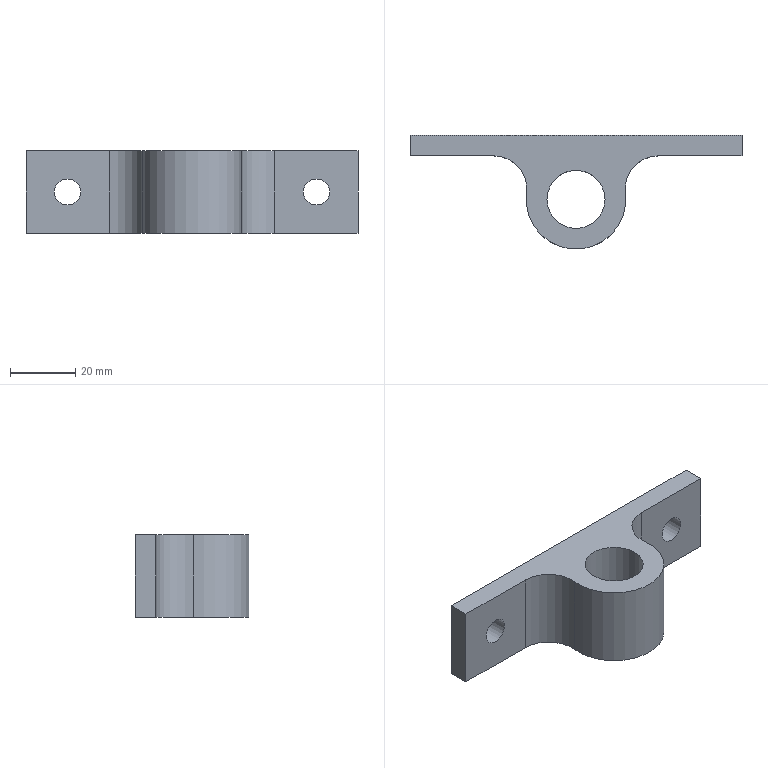Component | NX | BRACKET | 1 solid | 13 faces | box 101.6 x 34.93 x 25.4 mm | volume 30040 mm3 | plane 7 | cylinder 6 | commonest cylinder face diameters 20.32 x2 8 x2 30.48 x1 17.78 x1
STEP:
#1=CARTESIAN_POINT('',(0.,0.,0.));
#2=DIRECTION('',(0.,0.,1.));
#3=DIRECTION('',(1.,0.,0.));
#4=AXIS2_PLACEMENT_3D('',#1,#2,#3);
#5=CARTESIAN_POINT('',(50.8,13.335,627.));
#6=VERTEX_POINT('',#5);
#7=CARTESIAN_POINT('',(50.8,19.685,627.));
#8=VERTEX_POINT('',#7);
#9=CARTESIAN_POINT('',(50.8,13.335,627.));
#10=DIRECTION('',(0.,1.,0.));
#11=VECTOR('',#10,1.);
#12=LINE('',#9,#11);
#13=CARTESIAN_POINT('',(50.8,13.335,601.6));
#14=DIRECTION('',(1.,0.,0.));
#15=DIRECTION('',(0.,0.,1.));
#16=AXIS2_PLACEMENT_3D('',#13,#14,#15);
#17=PLANE('',#16);
#18=CARTESIAN_POINT('',(25.4,0.));
#19=DIRECTION('',(0.,-1.));
#20=VECTOR('',#19,1.);
#21=LINE('',#18,#20);
#22=(GEOMETRIC_REPRESENTATION_CONTEXT(2)PARAMETRIC_REPRESENTATION_CONTEXT()REPRESENTATION_CONTEXT('',''));
#23=DEFINITIONAL_REPRESENTATION('',(#21),#22);
#24=PCURVE('',#17,#23);
#25=CARTESIAN_POINT('',(-25.201,3.175,627.));
#26=DIRECTION('',(0.,0.,-1.));
#27=DIRECTION('',(1.,0.,0.));
#28=AXIS2_PLACEMENT_3D('',#25,#26,#27);
#29=PLANE('',#28);
#30=CARTESIAN_POINT('',(76.001,-10.16));
#31=DIRECTION('',(0.,-1.));
#32=VECTOR('',#31,1.);
#33=LINE('',#30,#32);
#34=(GEOMETRIC_REPRESENTATION_CONTEXT(2)PARAMETRIC_REPRESENTATION_CONTEXT()REPRESENTATION_CONTEXT('',''));
#35=DEFINITIONAL_REPRESENTATION('',(#33),#34);
#36=PCURVE('',#29,#35);
#37=SURFACE_CURVE('',#12,(#24,#36),.PCURVE_S1.);
#38=EDGE_CURVE('',#6,#8,#37,.T.);
#39=ORIENTED_EDGE('',*,*,#38,.F.);
#40=CARTESIAN_POINT('',(50.8,13.335,601.6));
#41=VERTEX_POINT('',#40);
#42=CARTESIAN_POINT('',(50.8,13.335,601.6));
#43=DIRECTION('',(0.,0.,1.));
#44=VECTOR('',#43,1.);
#45=LINE('',#42,#44);
#46=CARTESIAN_POINT('',(0.,0.));
#47=DIRECTION('',(1.,0.));
#48=VECTOR('',#47,1.);
#49=LINE('',#46,#48);
#50=(GEOMETRIC_REPRESENTATION_CONTEXT(2)PARAMETRIC_REPRESENTATION_CONTEXT()REPRESENTATION_CONTEXT('',''));
#51=DEFINITIONAL_REPRESENTATION('',(#49),#50);
#52=PCURVE('',#17,#51);
#53=CARTESIAN_POINT('',(25.201,13.335,601.6));
#54=DIRECTION('',(0.,-1.,0.));
#55=DIRECTION('',(1.,0.,0.));
#56=AXIS2_PLACEMENT_3D('',#53,#54,#55);
#57=PLANE('',#56);
#58=CARTESIAN_POINT('',(25.599,0.));
#59=DIRECTION('',(0.,1.));
#60=VECTOR('',#59,1.);
#61=LINE('',#58,#60);
#62=(GEOMETRIC_REPRESENTATION_CONTEXT(2)PARAMETRIC_REPRESENTATION_CONTEXT()REPRESENTATION_CONTEXT('',''));
#63=DEFINITIONAL_REPRESENTATION('',(#61),#62);
#64=PCURVE('',#57,#63);
#65=SURFACE_CURVE('',#45,(#52,#64),.PCURVE_S1.);
#66=EDGE_CURVE('',#41,#6,#65,.T.);
#67=ORIENTED_EDGE('',*,*,#66,.F.);
#68=CARTESIAN_POINT('',(50.8,19.685,601.6));
#69=VERTEX_POINT('',#68);
#70=CARTESIAN_POINT('',(50.8,13.335,601.6));
#71=DIRECTION('',(0.,1.,0.));
#72=VECTOR('',#71,1.);
#73=LINE('',#70,#72);
#74=CARTESIAN_POINT('',(0.,0.));
#75=DIRECTION('',(0.,-1.));
#76=VECTOR('',#75,1.);
#77=LINE('',#74,#76);
#78=(GEOMETRIC_REPRESENTATION_CONTEXT(2)PARAMETRIC_REPRESENTATION_CONTEXT()REPRESENTATION_CONTEXT('',''));
#79=DEFINITIONAL_REPRESENTATION('',(#77),#78);
#80=PCURVE('',#17,#79);
#81=CARTESIAN_POINT('',(-25.201,3.175,601.6));
#82=DIRECTION('',(0.,0.,-1.));
#83=DIRECTION('',(1.,0.,0.));
#84=AXIS2_PLACEMENT_3D('',#81,#82,#83);
#85=PLANE('',#84);
#86=CARTESIAN_POINT('',(76.001,-10.16));
#87=DIRECTION('',(0.,-1.));
#88=VECTOR('',#87,1.);
#89=LINE('',#86,#88);
#90=(GEOMETRIC_REPRESENTATION_CONTEXT(2)PARAMETRIC_REPRESENTATION_CONTEXT()REPRESENTATION_CONTEXT('',''));
#91=DEFINITIONAL_REPRESENTATION('',(#89),#90);
#92=PCURVE('',#85,#91);
#93=SURFACE_CURVE('',#73,(#80,#92),.PCURVE_S1.);
#94=EDGE_CURVE('',#41,#69,#93,.T.);
#95=ORIENTED_EDGE('',*,*,#94,.T.);
#96=CARTESIAN_POINT('',(50.8,19.685,601.6));
#97=DIRECTION('',(0.,0.,1.));
#98=VECTOR('',#97,1.);
#99=LINE('',#96,#98);
#100=CARTESIAN_POINT('',(0.,-6.35));
#101=DIRECTION('',(1.,0.));
#102=VECTOR('',#101,1.);
#103=LINE('',#100,#102);
#104=(GEOMETRIC_REPRESENTATION_CONTEXT(2)PARAMETRIC_REPRESENTATION_CONTEXT()REPRESENTATION_CONTEXT('',''));
#105=DEFINITIONAL_REPRESENTATION('',(#103),#104);
#106=PCURVE('',#17,#105);
#107=CARTESIAN_POINT('',(50.8,19.685,601.6));
#108=DIRECTION('',(-0.,1.,0.));
#109=DIRECTION('',(-1.,-0.,0.));
#110=AXIS2_PLACEMENT_3D('',#107,#108,#109);
#111=PLANE('',#110);
#112=CARTESIAN_POINT('',(0.,0.));
#113=DIRECTION('',(0.,1.));
#114=VECTOR('',#113,1.);
#115=LINE('',#112,#114);
#116=(GEOMETRIC_REPRESENTATION_CONTEXT(2)PARAMETRIC_REPRESENTATION_CONTEXT()REPRESENTATION_CONTEXT('',''));
#117=DEFINITIONAL_REPRESENTATION('',(#115),#116);
#118=PCURVE('',#111,#117);
#119=SURFACE_CURVE('',#99,(#106,#118),.PCURVE_S1.);
#120=EDGE_CURVE('',#69,#8,#119,.T.);
#121=ORIENTED_EDGE('',*,*,#120,.T.);
#122=EDGE_LOOP('',(#39,#67,#95,#121));
#123=FACE_BOUND('',#122,.T.);
#124=ADVANCED_FACE('',(#123),#17,.T.);
#125=CARTESIAN_POINT('',(34.1,19.685,614.3));
#126=VERTEX_POINT('',#125);
#127=CARTESIAN_POINT('',(38.1,19.685,614.3));
#128=DIRECTION('',(0.,-1.,0.));
#129=DIRECTION('',(-1.,-0.,0.));
#130=AXIS2_PLACEMENT_3D('',#127,#128,#129);
#131=CIRCLE('',#130,4.);
#132=CARTESIAN_POINT('',(16.7,12.7));
#133=CARTESIAN_POINT('',(16.7,5.772));
#134=CARTESIAN_POINT('',(10.7,9.236));
#135=CARTESIAN_POINT('',(4.7,12.7));
#136=CARTESIAN_POINT('',(10.7,16.164));
#137=CARTESIAN_POINT('',(16.7,19.628));
#138=CARTESIAN_POINT('',(16.7,12.7));
#139=(BOUNDED_CURVE()B_SPLINE_CURVE(2,(#132,#133,#134,#135,#136,#137,#138),.UNSPECIFIED.,.T.,.F.)B_SPLINE_CURVE_WITH_KNOTS((1,2,2,2,2,1),(-2.094,0.,2.094,4.189,6.283,8.378),.UNSPECIFIED.)CURVE()GEOMETRIC_REPRESENTATION_ITEM()RATIONAL_B_SPLINE_CURVE((1.,0.5,1.,0.5,1.,0.5,1.))REPRESENTATION_ITEM(''));
#140=(GEOMETRIC_REPRESENTATION_CONTEXT(2)PARAMETRIC_REPRESENTATION_CONTEXT()REPRESENTATION_CONTEXT('',''));
#141=DEFINITIONAL_REPRESENTATION('',(#139),#140);
#142=PCURVE('',#111,#141);
#143=CARTESIAN_POINT('',(38.1,38.735,614.3));
#144=DIRECTION('',(0.,-1.,0.));
#145=DIRECTION('',(0.,0.,1.));
#146=AXIS2_PLACEMENT_3D('',#143,#144,#145);
#147=CYLINDRICAL_SURFACE('',#146,4.);
#148=CARTESIAN_POINT('',(1.571,19.05));
#149=DIRECTION('',(1.,0.));
#150=VECTOR('',#149,1.);
#151=LINE('',#148,#150);
#152=(GEOMETRIC_REPRESENTATION_CONTEXT(2)PARAMETRIC_REPRESENTATION_CONTEXT()REPRESENTATION_CONTEXT('',''));
#153=DEFINITIONAL_REPRESENTATION('',(#151),#152);
#154=PCURVE('',#147,#153);
#155=SURFACE_CURVE('',#131,(#142,#154),.PCURVE_S1.);
#156=EDGE_CURVE('',#126,#126,#155,.T.);
#157=ORIENTED_EDGE('',*,*,#156,.T.);
#158=EDGE_LOOP('',(#157));
#159=FACE_BOUND('',#158,.T.);
#160=CARTESIAN_POINT('',(-42.1,19.685,614.3));
#161=VERTEX_POINT('',#160);
#162=CARTESIAN_POINT('',(-38.1,19.685,614.3));
#163=DIRECTION('',(-0.,1.,0.));
#164=DIRECTION('',(-1.,-0.,0.));
#165=AXIS2_PLACEMENT_3D('',#162,#163,#164);
#166=CIRCLE('',#165,4.);
#167=CARTESIAN_POINT('',(88.9,12.7));
#168=DIRECTION('',(1.,0.));
#169=AXIS2_PLACEMENT_2D('',#167,#168);
#170=CIRCLE('',#169,4.);
#171=(GEOMETRIC_REPRESENTATION_CONTEXT(2)PARAMETRIC_REPRESENTATION_CONTEXT()REPRESENTATION_CONTEXT('',''));
#172=DEFINITIONAL_REPRESENTATION('',(#170),#171);
#173=PCURVE('',#111,#172);
#174=CARTESIAN_POINT('',(-38.1,38.735,614.3));
#175=DIRECTION('',(0.,-1.,0.));
#176=DIRECTION('',(0.,0.,1.));
#177=AXIS2_PLACEMENT_3D('',#174,#175,#176);
#178=CYLINDRICAL_SURFACE('',#177,4.);
#179=CARTESIAN_POINT('',(7.854,19.05));
#180=DIRECTION('',(-1.,0.));
#181=VECTOR('',#180,1.);
#182=LINE('',#179,#181);
#183=(GEOMETRIC_REPRESENTATION_CONTEXT(2)PARAMETRIC_REPRESENTATION_CONTEXT()REPRESENTATION_CONTEXT('',''));
#184=DEFINITIONAL_REPRESENTATION('',(#182),#183);
#185=PCURVE('',#178,#184);
#186=SURFACE_CURVE('',#166,(#173,#185),.PCURVE_S1.);
#187=EDGE_CURVE('',#161,#161,#186,.T.);
#188=ORIENTED_EDGE('',*,*,#187,.F.);
#189=EDGE_LOOP('',(#188));
#190=FACE_BOUND('',#189,.T.);
#191=CARTESIAN_POINT('',(-50.8,19.685,627.));
#192=VERTEX_POINT('',#191);
#193=CARTESIAN_POINT('',(50.8,19.685,627.));
#194=DIRECTION('',(-1.,-0.,0.));
#195=VECTOR('',#194,1.);
#196=LINE('',#193,#195);
#197=CARTESIAN_POINT('',(0.,25.4));
#198=DIRECTION('',(1.,0.));
#199=VECTOR('',#198,1.);
#200=LINE('',#197,#199);
#201=(GEOMETRIC_REPRESENTATION_CONTEXT(2)PARAMETRIC_REPRESENTATION_CONTEXT()REPRESENTATION_CONTEXT('',''));
#202=DEFINITIONAL_REPRESENTATION('',(#200),#201);
#203=PCURVE('',#111,#202);
#204=CARTESIAN_POINT('',(76.001,-16.51));
#205=DIRECTION('',(-1.,0.));
#206=VECTOR('',#205,1.);
#207=LINE('',#204,#206);
#208=(GEOMETRIC_REPRESENTATION_CONTEXT(2)PARAMETRIC_REPRESENTATION_CONTEXT()REPRESENTATION_CONTEXT('',''));
#209=DEFINITIONAL_REPRESENTATION('',(#207),#208);
#210=PCURVE('',#29,#209);
#211=SURFACE_CURVE('',#196,(#203,#210),.PCURVE_S1.);
#212=EDGE_CURVE('',#8,#192,#211,.T.);
#213=ORIENTED_EDGE('',*,*,#212,.F.);
#214=ORIENTED_EDGE('',*,*,#120,.F.);
#215=CARTESIAN_POINT('',(-50.8,19.685,601.6));
#216=VERTEX_POINT('',#215);
#217=CARTESIAN_POINT('',(50.8,19.685,601.6));
#218=DIRECTION('',(-1.,-0.,0.));
#219=VECTOR('',#218,1.);
#220=LINE('',#217,#219);
#221=CARTESIAN_POINT('',(0.,0.));
#222=DIRECTION('',(1.,0.));
#223=VECTOR('',#222,1.);
#224=LINE('',#221,#223);
#225=(GEOMETRIC_REPRESENTATION_CONTEXT(2)PARAMETRIC_REPRESENTATION_CONTEXT()REPRESENTATION_CONTEXT('',''));
#226=DEFINITIONAL_REPRESENTATION('',(#224),#225);
#227=PCURVE('',#111,#226);
#228=CARTESIAN_POINT('',(76.001,-16.51));
#229=DIRECTION('',(-1.,0.));
#230=VECTOR('',#229,1.);
#231=LINE('',#228,#230);
#232=(GEOMETRIC_REPRESENTATION_CONTEXT(2)PARAMETRIC_REPRESENTATION_CONTEXT()REPRESENTATION_CONTEXT('',''));
#233=DEFINITIONAL_REPRESENTATION('',(#231),#232);
#234=PCURVE('',#85,#233);
#235=SURFACE_CURVE('',#220,(#227,#234),.PCURVE_S1.);
#236=EDGE_CURVE('',#69,#216,#235,.T.);
#237=ORIENTED_EDGE('',*,*,#236,.T.);
#238=CARTESIAN_POINT('',(-50.8,19.685,601.6));
#239=DIRECTION('',(0.,0.,1.));
#240=VECTOR('',#239,1.);
#241=LINE('',#238,#240);
#242=CARTESIAN_POINT('',(101.6,0.));
#243=DIRECTION('',(0.,1.));
#244=VECTOR('',#243,1.);
#245=LINE('',#242,#244);
#246=(GEOMETRIC_REPRESENTATION_CONTEXT(2)PARAMETRIC_REPRESENTATION_CONTEXT()REPRESENTATION_CONTEXT('',''));
#247=DEFINITIONAL_REPRESENTATION('',(#245),#246);
#248=PCURVE('',#111,#247);
#249=CARTESIAN_POINT('',(-50.8,19.685,601.6));
#250=DIRECTION('',(-1.,0.,0.));
#251=DIRECTION('',(0.,0.,-1.));
#252=AXIS2_PLACEMENT_3D('',#249,#250,#251);
#253=PLANE('',#252);
#254=CARTESIAN_POINT('',(0.,0.));
#255=DIRECTION('',(-1.,0.));
#256=VECTOR('',#255,1.);
#257=LINE('',#254,#256);
#258=(GEOMETRIC_REPRESENTATION_CONTEXT(2)PARAMETRIC_REPRESENTATION_CONTEXT()REPRESENTATION_CONTEXT('',''));
#259=DEFINITIONAL_REPRESENTATION('',(#257),#258);
#260=PCURVE('',#253,#259);
#261=SURFACE_CURVE('',#241,(#248,#260),.PCURVE_S1.);
#262=EDGE_CURVE('',#216,#192,#261,.T.);
#263=ORIENTED_EDGE('',*,*,#262,.T.);
#264=EDGE_LOOP('',(#213,#214,#237,#263));
#265=FACE_BOUND('',#264,.T.);
#266=ADVANCED_FACE('',(#159,#190,#265),#111,.T.);
#267=CARTESIAN_POINT('',(-50.8,13.335,627.));
#268=VERTEX_POINT('',#267);
#269=CARTESIAN_POINT('',(-50.8,19.685,627.));
#270=DIRECTION('',(0.,-1.,0.));
#271=VECTOR('',#270,1.);
#272=LINE('',#269,#271);
#273=CARTESIAN_POINT('',(-25.4,0.));
#274=DIRECTION('',(0.,1.));
#275=VECTOR('',#274,1.);
#276=LINE('',#273,#275);
#277=(GEOMETRIC_REPRESENTATION_CONTEXT(2)PARAMETRIC_REPRESENTATION_CONTEXT()REPRESENTATION_CONTEXT('',''));
#278=DEFINITIONAL_REPRESENTATION('',(#276),#277);
#279=PCURVE('',#253,#278);
#280=CARTESIAN_POINT('',(-25.599,-16.51));
#281=DIRECTION('',(0.,1.));
#282=VECTOR('',#281,1.);
#283=LINE('',#280,#282);
#284=(GEOMETRIC_REPRESENTATION_CONTEXT(2)PARAMETRIC_REPRESENTATION_CONTEXT()REPRESENTATION_CONTEXT('',''));
#285=DEFINITIONAL_REPRESENTATION('',(#283),#284);
#286=PCURVE('',#29,#285);
#287=SURFACE_CURVE('',#272,(#279,#286),.PCURVE_S1.);
#288=EDGE_CURVE('',#192,#268,#287,.T.);
#289=ORIENTED_EDGE('',*,*,#288,.F.);
#290=ORIENTED_EDGE('',*,*,#262,.F.);
#291=CARTESIAN_POINT('',(-50.8,13.335,601.6));
#292=VERTEX_POINT('',#291);
#293=CARTESIAN_POINT('',(-50.8,19.685,601.6));
#294=DIRECTION('',(0.,-1.,0.));
#295=VECTOR('',#294,1.);
#296=LINE('',#293,#295);
#297=CARTESIAN_POINT('',(0.,0.));
#298=DIRECTION('',(0.,1.));
#299=VECTOR('',#298,1.);
#300=LINE('',#297,#299);
#301=(GEOMETRIC_REPRESENTATION_CONTEXT(2)PARAMETRIC_REPRESENTATION_CONTEXT()REPRESENTATION_CONTEXT('',''));
#302=DEFINITIONAL_REPRESENTATION('',(#300),#301);
#303=PCURVE('',#253,#302);
#304=CARTESIAN_POINT('',(-25.599,-16.51));
#305=DIRECTION('',(0.,1.));
#306=VECTOR('',#305,1.);
#307=LINE('',#304,#306);
#308=(GEOMETRIC_REPRESENTATION_CONTEXT(2)PARAMETRIC_REPRESENTATION_CONTEXT()REPRESENTATION_CONTEXT('',''));
#309=DEFINITIONAL_REPRESENTATION('',(#307),#308);
#310=PCURVE('',#85,#309);
#311=SURFACE_CURVE('',#296,(#303,#310),.PCURVE_S1.);
#312=EDGE_CURVE('',#216,#292,#311,.T.);
#313=ORIENTED_EDGE('',*,*,#312,.T.);
#314=CARTESIAN_POINT('',(-50.8,13.335,601.6));
#315=DIRECTION('',(0.,0.,1.));
#316=VECTOR('',#315,1.);
#317=LINE('',#314,#316);
#318=CARTESIAN_POINT('',(0.,6.35));
#319=DIRECTION('',(-1.,0.));
#320=VECTOR('',#319,1.);
#321=LINE('',#318,#320);
#322=(GEOMETRIC_REPRESENTATION_CONTEXT(2)PARAMETRIC_REPRESENTATION_CONTEXT()REPRESENTATION_CONTEXT('',''));
#323=DEFINITIONAL_REPRESENTATION('',(#321),#322);
#324=PCURVE('',#253,#323);
#325=CARTESIAN_POINT('',(-50.8,13.335,601.6));
#326=DIRECTION('',(0.,-1.,0.));
#327=DIRECTION('',(1.,0.,0.));
#328=AXIS2_PLACEMENT_3D('',#325,#326,#327);
#329=PLANE('',#328);
#330=CARTESIAN_POINT('',(0.,0.));
#331=DIRECTION('',(0.,1.));
#332=VECTOR('',#331,1.);
#333=LINE('',#330,#332);
#334=(GEOMETRIC_REPRESENTATION_CONTEXT(2)PARAMETRIC_REPRESENTATION_CONTEXT()REPRESENTATION_CONTEXT('',''));
#335=DEFINITIONAL_REPRESENTATION('',(#333),#334);
#336=PCURVE('',#329,#335);
#337=SURFACE_CURVE('',#317,(#324,#336),.PCURVE_S1.);
#338=EDGE_CURVE('',#292,#268,#337,.T.);
#339=ORIENTED_EDGE('',*,*,#338,.T.);
#340=EDGE_LOOP('',(#289,#290,#313,#339));
#341=FACE_BOUND('',#340,.T.);
#342=ADVANCED_FACE('',(#341),#253,.T.);
#343=CARTESIAN_POINT('',(-42.1,13.335,614.3));
#344=VERTEX_POINT('',#343);
#345=CARTESIAN_POINT('',(-38.1,13.335,614.3));
#346=DIRECTION('',(-0.,-1.,0.));
#347=DIRECTION('',(-1.,0.,0.));
#348=AXIS2_PLACEMENT_3D('',#345,#346,#347);
#349=CIRCLE('',#348,4.);
#350=CARTESIAN_POINT('',(12.7,12.7));
#351=DIRECTION('',(-1.,0.));
#352=AXIS2_PLACEMENT_2D('',#350,#351);
#353=CIRCLE('',#352,4.);
#354=(GEOMETRIC_REPRESENTATION_CONTEXT(2)PARAMETRIC_REPRESENTATION_CONTEXT()REPRESENTATION_CONTEXT('',''));
#355=DEFINITIONAL_REPRESENTATION('',(#353),#354);
#356=PCURVE('',#329,#355);
#357=CARTESIAN_POINT('',(1.571,25.4));
#358=DIRECTION('',(1.,0.));
#359=VECTOR('',#358,1.);
#360=LINE('',#357,#359);
#361=(GEOMETRIC_REPRESENTATION_CONTEXT(2)PARAMETRIC_REPRESENTATION_CONTEXT()REPRESENTATION_CONTEXT('',''));
#362=DEFINITIONAL_REPRESENTATION('',(#360),#361);
#363=PCURVE('',#178,#362);
#364=SURFACE_CURVE('',#349,(#356,#363),.PCURVE_S1.);
#365=EDGE_CURVE('',#344,#344,#364,.T.);
#366=ORIENTED_EDGE('',*,*,#365,.F.);
#367=EDGE_LOOP('',(#366));
#368=FACE_BOUND('',#367,.T.);
#369=CARTESIAN_POINT('',(-25.201,13.335,627.));
#370=VERTEX_POINT('',#369);
#371=CARTESIAN_POINT('',(-50.8,13.335,627.));
#372=DIRECTION('',(1.,0.,0.));
#373=VECTOR('',#372,1.);
#374=LINE('',#371,#373);
#375=CARTESIAN_POINT('',(0.,25.4));
#376=DIRECTION('',(1.,0.));
#377=VECTOR('',#376,1.);
#378=LINE('',#375,#377);
#379=(GEOMETRIC_REPRESENTATION_CONTEXT(2)PARAMETRIC_REPRESENTATION_CONTEXT()REPRESENTATION_CONTEXT('',''));
#380=DEFINITIONAL_REPRESENTATION('',(#378),#379);
#381=PCURVE('',#329,#380);
#382=CARTESIAN_POINT('',(-25.599,-10.16));
#383=DIRECTION('',(1.,-0.));
#384=VECTOR('',#383,1.);
#385=LINE('',#382,#384);
#386=(GEOMETRIC_REPRESENTATION_CONTEXT(2)PARAMETRIC_REPRESENTATION_CONTEXT()REPRESENTATION_CONTEXT('',''));
#387=DEFINITIONAL_REPRESENTATION('',(#385),#386);
#388=PCURVE('',#29,#387);
#389=SURFACE_CURVE('',#374,(#381,#388),.PCURVE_S1.);
#390=EDGE_CURVE('',#268,#370,#389,.T.);
#391=ORIENTED_EDGE('',*,*,#390,.F.);
#392=ORIENTED_EDGE('',*,*,#338,.F.);
#393=CARTESIAN_POINT('',(-25.201,13.335,601.6));
#394=VERTEX_POINT('',#393);
#395=CARTESIAN_POINT('',(-50.8,13.335,601.6));
#396=DIRECTION('',(1.,0.,0.));
#397=VECTOR('',#396,1.);
#398=LINE('',#395,#397);
#399=CARTESIAN_POINT('',(0.,0.));
#400=DIRECTION('',(1.,0.));
#401=VECTOR('',#400,1.);
#402=LINE('',#399,#401);
#403=(GEOMETRIC_REPRESENTATION_CONTEXT(2)PARAMETRIC_REPRESENTATION_CONTEXT()REPRESENTATION_CONTEXT('',''));
#404=DEFINITIONAL_REPRESENTATION('',(#402),#403);
#405=PCURVE('',#329,#404);
#406=CARTESIAN_POINT('',(-25.599,-10.16));
#407=DIRECTION('',(1.,-0.));
#408=VECTOR('',#407,1.);
#409=LINE('',#406,#408);
#410=(GEOMETRIC_REPRESENTATION_CONTEXT(2)PARAMETRIC_REPRESENTATION_CONTEXT()REPRESENTATION_CONTEXT('',''));
#411=DEFINITIONAL_REPRESENTATION('',(#409),#410);
#412=PCURVE('',#85,#411);
#413=SURFACE_CURVE('',#398,(#405,#412),.PCURVE_S1.);
#414=EDGE_CURVE('',#292,#394,#413,.T.);
#415=ORIENTED_EDGE('',*,*,#414,.T.);
#416=CARTESIAN_POINT('',(-25.201,13.335,601.6));
#417=DIRECTION('',(0.,0.,1.));
#418=VECTOR('',#417,1.);
#419=LINE('',#416,#418);
#420=CARTESIAN_POINT('',(25.599,0.));
#421=DIRECTION('',(0.,1.));
#422=VECTOR('',#421,1.);
#423=LINE('',#420,#422);
#424=(GEOMETRIC_REPRESENTATION_CONTEXT(2)PARAMETRIC_REPRESENTATION_CONTEXT()REPRESENTATION_CONTEXT('',''));
#425=DEFINITIONAL_REPRESENTATION('',(#423),#424);
#426=PCURVE('',#329,#425);
#427=CARTESIAN_POINT('',(-25.201,3.175,601.6));
#428=DIRECTION('',(0.,0.,1.));
#429=DIRECTION('',(-1.,0.,0.));
#430=AXIS2_PLACEMENT_3D('',#427,#428,#429);
#431=CYLINDRICAL_SURFACE('',#430,10.16);
#432=CARTESIAN_POINT('',(4.712,0.));
#433=DIRECTION('',(0.,1.));
#434=VECTOR('',#433,1.);
#435=LINE('',#432,#434);
#436=(GEOMETRIC_REPRESENTATION_CONTEXT(2)PARAMETRIC_REPRESENTATION_CONTEXT()REPRESENTATION_CONTEXT('',''));
#437=DEFINITIONAL_REPRESENTATION('',(#435),#436);
#438=PCURVE('',#431,#437);
#439=SURFACE_CURVE('',#419,(#426,#438),.PCURVE_S1.);
#440=EDGE_CURVE('',#394,#370,#439,.T.);
#441=ORIENTED_EDGE('',*,*,#440,.T.);
#442=EDGE_LOOP('',(#391,#392,#415,#441));
#443=FACE_BOUND('',#442,.T.);
#444=ADVANCED_FACE('',(#368,#443),#329,.T.);
#445=CARTESIAN_POINT('',(-15.12,1.905,601.6));
#446=VERTEX_POINT('',#445);
#447=CARTESIAN_POINT('',(-15.12,1.905,627.));
#448=VERTEX_POINT('',#447);
#449=CARTESIAN_POINT('',(-15.12,1.905,601.6));
#450=DIRECTION('',(0.,0.,1.));
#451=VECTOR('',#450,1.);
#452=LINE('',#449,#451);
#453=CARTESIAN_POINT('',(3.016,0.));
#454=DIRECTION('',(0.,1.));
#455=VECTOR('',#454,1.);
#456=LINE('',#453,#455);
#457=(GEOMETRIC_REPRESENTATION_CONTEXT(2)PARAMETRIC_REPRESENTATION_CONTEXT()REPRESENTATION_CONTEXT('',''));
#458=DEFINITIONAL_REPRESENTATION('',(#456),#457);
#459=PCURVE('',#431,#458);
#460=CARTESIAN_POINT('',(0.,-0.,601.6));
#461=DIRECTION('',(0.,0.,1.));
#462=DIRECTION('',(-1.,0.,0.));
#463=AXIS2_PLACEMENT_3D('',#460,#461,#462);
#464=CYLINDRICAL_SURFACE('',#463,15.24);
#465=CARTESIAN_POINT('',(-0.1253,0.));
#466=DIRECTION('',(0.,1.));
#467=VECTOR('',#466,1.);
#468=LINE('',#465,#467);
#469=(GEOMETRIC_REPRESENTATION_CONTEXT(2)PARAMETRIC_REPRESENTATION_CONTEXT()REPRESENTATION_CONTEXT('',''));
#470=DEFINITIONAL_REPRESENTATION('',(#468),#469);
#471=PCURVE('',#464,#470);
#472=SURFACE_CURVE('',#452,(#459,#471),.PCURVE_S1.);
#473=EDGE_CURVE('',#446,#448,#472,.T.);
#474=ORIENTED_EDGE('',*,*,#473,.F.);
#475=CARTESIAN_POINT('',(-25.201,3.175,601.6));
#476=DIRECTION('',(0.,0.,-1.));
#477=DIRECTION('',(1.,0.,0.));
#478=AXIS2_PLACEMENT_3D('',#475,#476,#477);
#479=CIRCLE('',#478,10.16);
#480=CARTESIAN_POINT('',(9.425,0.));
#481=DIRECTION('',(-1.,0.));
#482=VECTOR('',#481,1.);
#483=LINE('',#480,#482);
#484=(GEOMETRIC_REPRESENTATION_CONTEXT(2)PARAMETRIC_REPRESENTATION_CONTEXT()REPRESENTATION_CONTEXT('',''));
#485=DEFINITIONAL_REPRESENTATION('',(#483),#484);
#486=PCURVE('',#431,#485);
#487=CARTESIAN_POINT('',(0.,0.));
#488=DIRECTION('',(1.,0.));
#489=AXIS2_PLACEMENT_2D('',#487,#488);
#490=CIRCLE('',#489,10.16);
#491=(GEOMETRIC_REPRESENTATION_CONTEXT(2)PARAMETRIC_REPRESENTATION_CONTEXT()REPRESENTATION_CONTEXT('',''));
#492=DEFINITIONAL_REPRESENTATION('',(#490),#491);
#493=PCURVE('',#85,#492);
#494=SURFACE_CURVE('',#479,(#486,#493),.PCURVE_S1.);
#495=EDGE_CURVE('',#394,#446,#494,.T.);
#496=ORIENTED_EDGE('',*,*,#495,.F.);
#497=ORIENTED_EDGE('',*,*,#440,.T.);
#498=CARTESIAN_POINT('',(-25.201,3.175,627.));
#499=DIRECTION('',(0.,0.,-1.));
#500=DIRECTION('',(1.,0.,0.));
#501=AXIS2_PLACEMENT_3D('',#498,#499,#500);
#502=CIRCLE('',#501,10.16);
#503=CARTESIAN_POINT('',(9.425,25.4));
#504=DIRECTION('',(-1.,0.));
#505=VECTOR('',#504,1.);
#506=LINE('',#503,#505);
#507=(GEOMETRIC_REPRESENTATION_CONTEXT(2)PARAMETRIC_REPRESENTATION_CONTEXT()REPRESENTATION_CONTEXT('',''));
#508=DEFINITIONAL_REPRESENTATION('',(#506),#507);
#509=PCURVE('',#431,#508);
#510=CARTESIAN_POINT('',(0.,0.));
#511=DIRECTION('',(1.,0.));
#512=AXIS2_PLACEMENT_2D('',#510,#511);
#513=CIRCLE('',#512,10.16);
#514=(GEOMETRIC_REPRESENTATION_CONTEXT(2)PARAMETRIC_REPRESENTATION_CONTEXT()REPRESENTATION_CONTEXT('',''));
#515=DEFINITIONAL_REPRESENTATION('',(#513),#514);
#516=PCURVE('',#29,#515);
#517=SURFACE_CURVE('',#502,(#509,#516),.PCURVE_S1.);
#518=EDGE_CURVE('',#370,#448,#517,.T.);
#519=ORIENTED_EDGE('',*,*,#518,.T.);
#520=EDGE_LOOP('',(#474,#496,#497,#519));
#521=FACE_BOUND('',#520,.F.);
#522=ADVANCED_FACE('',(#521),#431,.F.);
#523=CARTESIAN_POINT('',(15.12,1.905,627.));
#524=VERTEX_POINT('',#523);
#525=CARTESIAN_POINT('',(0.,-0.,627.));
#526=DIRECTION('',(0.,0.,1.));
#527=DIRECTION('',(1.,-0.,0.));
#528=AXIS2_PLACEMENT_3D('',#525,#526,#527);
#529=CIRCLE('',#528,15.24);
#530=CARTESIAN_POINT('',(-3.142,25.4));
#531=DIRECTION('',(1.,0.));
#532=VECTOR('',#531,1.);
#533=LINE('',#530,#532);
#534=(GEOMETRIC_REPRESENTATION_CONTEXT(2)PARAMETRIC_REPRESENTATION_CONTEXT()REPRESENTATION_CONTEXT('',''));
#535=DEFINITIONAL_REPRESENTATION('',(#533),#534);
#536=PCURVE('',#464,#535);
#537=CARTESIAN_POINT('',(40.441,3.175));
#538=CARTESIAN_POINT('',(40.441,-23.221));
#539=CARTESIAN_POINT('',(17.581,-10.023));
#540=CARTESIAN_POINT('',(-5.279,3.175));
#541=CARTESIAN_POINT('',(17.581,16.373));
#542=CARTESIAN_POINT('',(40.441,29.571));
#543=CARTESIAN_POINT('',(40.441,3.175));
#544=(BOUNDED_CURVE()B_SPLINE_CURVE(2,(#537,#538,#539,#540,#541,#542,#543),.UNSPECIFIED.,.T.,.F.)B_SPLINE_CURVE_WITH_KNOTS((1,2,2,2,2,1),(-2.094,0.,2.094,4.189,6.283,8.378),.UNSPECIFIED.)CURVE()GEOMETRIC_REPRESENTATION_ITEM()RATIONAL_B_SPLINE_CURVE((1.,0.5,1.,0.5,1.,0.5,1.))REPRESENTATION_ITEM(''));
#545=(GEOMETRIC_REPRESENTATION_CONTEXT(2)PARAMETRIC_REPRESENTATION_CONTEXT()REPRESENTATION_CONTEXT('',''));
#546=DEFINITIONAL_REPRESENTATION('',(#544),#545);
#547=PCURVE('',#29,#546);
#548=SURFACE_CURVE('',#529,(#536,#547),.PCURVE_S1.);
#549=EDGE_CURVE('',#448,#524,#548,.T.);
#550=ORIENTED_EDGE('',*,*,#549,.F.);
#551=ORIENTED_EDGE('',*,*,#473,.F.);
#552=CARTESIAN_POINT('',(15.12,1.905,601.6));
#553=VERTEX_POINT('',#552);
#554=CARTESIAN_POINT('',(0.,-0.,601.6));
#555=DIRECTION('',(0.,0.,1.));
#556=DIRECTION('',(1.,-0.,0.));
#557=AXIS2_PLACEMENT_3D('',#554,#555,#556);
#558=CIRCLE('',#557,15.24);
#559=CARTESIAN_POINT('',(-3.142,0.));
#560=DIRECTION('',(1.,0.));
#561=VECTOR('',#560,1.);
#562=LINE('',#559,#561);
#563=(GEOMETRIC_REPRESENTATION_CONTEXT(2)PARAMETRIC_REPRESENTATION_CONTEXT()REPRESENTATION_CONTEXT('',''));
#564=DEFINITIONAL_REPRESENTATION('',(#562),#563);
#565=PCURVE('',#464,#564);
#566=CARTESIAN_POINT('',(40.441,3.175));
#567=CARTESIAN_POINT('',(40.441,-23.221));
#568=CARTESIAN_POINT('',(17.581,-10.023));
#569=CARTESIAN_POINT('',(-5.279,3.175));
#570=CARTESIAN_POINT('',(17.581,16.373));
#571=CARTESIAN_POINT('',(40.441,29.571));
#572=CARTESIAN_POINT('',(40.441,3.175));
#573=(BOUNDED_CURVE()B_SPLINE_CURVE(2,(#566,#567,#568,#569,#570,#571,#572),.UNSPECIFIED.,.T.,.F.)B_SPLINE_CURVE_WITH_KNOTS((1,2,2,2,2,1),(-2.094,0.,2.094,4.189,6.283,8.378),.UNSPECIFIED.)CURVE()GEOMETRIC_REPRESENTATION_ITEM()RATIONAL_B_SPLINE_CURVE((1.,0.5,1.,0.5,1.,0.5,1.))REPRESENTATION_ITEM(''));
#574=(GEOMETRIC_REPRESENTATION_CONTEXT(2)PARAMETRIC_REPRESENTATION_CONTEXT()REPRESENTATION_CONTEXT('',''));
#575=DEFINITIONAL_REPRESENTATION('',(#573),#574);
#576=PCURVE('',#85,#575);
#577=SURFACE_CURVE('',#558,(#565,#576),.PCURVE_S1.);
#578=EDGE_CURVE('',#446,#553,#577,.T.);
#579=ORIENTED_EDGE('',*,*,#578,.T.);
#580=CARTESIAN_POINT('',(15.12,1.905,601.6));
#581=DIRECTION('',(0.,0.,1.));
#582=VECTOR('',#581,1.);
#583=LINE('',#580,#582);
#584=CARTESIAN_POINT('',(3.267,0.));
#585=DIRECTION('',(0.,1.));
#586=VECTOR('',#585,1.);
#587=LINE('',#584,#586);
#588=(GEOMETRIC_REPRESENTATION_CONTEXT(2)PARAMETRIC_REPRESENTATION_CONTEXT()REPRESENTATION_CONTEXT('',''));
#589=DEFINITIONAL_REPRESENTATION('',(#587),#588);
#590=PCURVE('',#464,#589);
#591=CARTESIAN_POINT('',(25.201,3.175,601.6));
#592=DIRECTION('',(0.,0.,1.));
#593=DIRECTION('',(-1.,0.,0.));
#594=AXIS2_PLACEMENT_3D('',#591,#592,#593);
#595=CYLINDRICAL_SURFACE('',#594,10.16);
#596=CARTESIAN_POINT('',(6.409,0.));
#597=DIRECTION('',(0.,1.));
#598=VECTOR('',#597,1.);
#599=LINE('',#596,#598);
#600=(GEOMETRIC_REPRESENTATION_CONTEXT(2)PARAMETRIC_REPRESENTATION_CONTEXT()REPRESENTATION_CONTEXT('',''));
#601=DEFINITIONAL_REPRESENTATION('',(#599),#600);
#602=PCURVE('',#595,#601);
#603=SURFACE_CURVE('',#583,(#590,#602),.PCURVE_S1.);
#604=EDGE_CURVE('',#553,#524,#603,.T.);
#605=ORIENTED_EDGE('',*,*,#604,.T.);
#606=EDGE_LOOP('',(#550,#551,#579,#605));
#607=FACE_BOUND('',#606,.T.);
#608=ADVANCED_FACE('',(#607),#464,.T.);
#609=CARTESIAN_POINT('',(25.201,13.335,601.6));
#610=VERTEX_POINT('',#609);
#611=CARTESIAN_POINT('',(25.201,13.335,627.));
#612=VERTEX_POINT('',#611);
#613=CARTESIAN_POINT('',(25.201,13.335,601.6));
#614=DIRECTION('',(0.,0.,1.));
#615=VECTOR('',#614,1.);
#616=LINE('',#613,#615);
#617=CARTESIAN_POINT('',(4.712,0.));
#618=DIRECTION('',(0.,1.));
#619=VECTOR('',#618,1.);
#620=LINE('',#617,#619);
#621=(GEOMETRIC_REPRESENTATION_CONTEXT(2)PARAMETRIC_REPRESENTATION_CONTEXT()REPRESENTATION_CONTEXT('',''));
#622=DEFINITIONAL_REPRESENTATION('',(#620),#621);
#623=PCURVE('',#595,#622);
#624=CARTESIAN_POINT('',(0.,0.));
#625=DIRECTION('',(0.,1.));
#626=VECTOR('',#625,1.);
#627=LINE('',#624,#626);
#628=(GEOMETRIC_REPRESENTATION_CONTEXT(2)PARAMETRIC_REPRESENTATION_CONTEXT()REPRESENTATION_CONTEXT('',''));
#629=DEFINITIONAL_REPRESENTATION('',(#627),#628);
#630=PCURVE('',#57,#629);
#631=SURFACE_CURVE('',#616,(#623,#630),.PCURVE_S1.);
#632=EDGE_CURVE('',#610,#612,#631,.T.);
#633=ORIENTED_EDGE('',*,*,#632,.F.);
#634=CARTESIAN_POINT('',(25.201,3.175,601.6));
#635=DIRECTION('',(0.,0.,-1.));
#636=DIRECTION('',(1.,0.,0.));
#637=AXIS2_PLACEMENT_3D('',#634,#635,#636);
#638=CIRCLE('',#637,10.16);
#639=CARTESIAN_POINT('',(9.425,0.));
#640=DIRECTION('',(-1.,0.));
#641=VECTOR('',#640,1.);
#642=LINE('',#639,#641);
#643=(GEOMETRIC_REPRESENTATION_CONTEXT(2)PARAMETRIC_REPRESENTATION_CONTEXT()REPRESENTATION_CONTEXT('',''));
#644=DEFINITIONAL_REPRESENTATION('',(#642),#643);
#645=PCURVE('',#595,#644);
#646=CARTESIAN_POINT('',(50.402,-0.));
#647=DIRECTION('',(1.,0.));
#648=AXIS2_PLACEMENT_2D('',#646,#647);
#649=CIRCLE('',#648,10.16);
#650=(GEOMETRIC_REPRESENTATION_CONTEXT(2)PARAMETRIC_REPRESENTATION_CONTEXT()REPRESENTATION_CONTEXT('',''));
#651=DEFINITIONAL_REPRESENTATION('',(#649),#650);
#652=PCURVE('',#85,#651);
#653=SURFACE_CURVE('',#638,(#645,#652),.PCURVE_S1.);
#654=EDGE_CURVE('',#553,#610,#653,.T.);
#655=ORIENTED_EDGE('',*,*,#654,.F.);
#656=ORIENTED_EDGE('',*,*,#604,.T.);
#657=CARTESIAN_POINT('',(25.201,3.175,627.));
#658=DIRECTION('',(0.,0.,-1.));
#659=DIRECTION('',(1.,0.,0.));
#660=AXIS2_PLACEMENT_3D('',#657,#658,#659);
#661=CIRCLE('',#660,10.16);
#662=CARTESIAN_POINT('',(9.425,25.4));
#663=DIRECTION('',(-1.,0.));
#664=VECTOR('',#663,1.);
#665=LINE('',#662,#664);
#666=(GEOMETRIC_REPRESENTATION_CONTEXT(2)PARAMETRIC_REPRESENTATION_CONTEXT()REPRESENTATION_CONTEXT('',''));
#667=DEFINITIONAL_REPRESENTATION('',(#665),#666);
#668=PCURVE('',#595,#667);
#669=CARTESIAN_POINT('',(50.402,-0.));
#670=DIRECTION('',(1.,0.));
#671=AXIS2_PLACEMENT_2D('',#669,#670);
#672=CIRCLE('',#671,10.16);
#673=(GEOMETRIC_REPRESENTATION_CONTEXT(2)PARAMETRIC_REPRESENTATION_CONTEXT()REPRESENTATION_CONTEXT('',''));
#674=DEFINITIONAL_REPRESENTATION('',(#672),#673);
#675=PCURVE('',#29,#674);
#676=SURFACE_CURVE('',#661,(#668,#675),.PCURVE_S1.);
#677=EDGE_CURVE('',#524,#612,#676,.T.);
#678=ORIENTED_EDGE('',*,*,#677,.T.);
#679=EDGE_LOOP('',(#633,#655,#656,#678));
#680=FACE_BOUND('',#679,.F.);
#681=ADVANCED_FACE('',(#680),#595,.F.);
#682=CARTESIAN_POINT('',(42.1,13.335,614.3));
#683=VERTEX_POINT('',#682);
#684=CARTESIAN_POINT('',(34.1,13.335,614.3));
#685=VERTEX_POINT('',#684);
#686=CARTESIAN_POINT('',(38.1,13.335,614.3));
#687=DIRECTION('',(-0.,1.,0.));
#688=DIRECTION('',(1.,0.,0.));
#689=AXIS2_PLACEMENT_3D('',#686,#687,#688);
#690=CIRCLE('',#689,4.);
#691=CARTESIAN_POINT('',(16.899,12.7));
#692=CARTESIAN_POINT('',(16.899,5.772));
#693=CARTESIAN_POINT('',(10.899,9.236));
#694=CARTESIAN_POINT('',(4.899,12.7));
#695=CARTESIAN_POINT('',(10.899,16.164));
#696=CARTESIAN_POINT('',(16.899,19.628));
#697=CARTESIAN_POINT('',(16.899,12.7));
#698=(BOUNDED_CURVE()B_SPLINE_CURVE(2,(#691,#692,#693,#694,#695,#696,#697),.UNSPECIFIED.,.T.,.F.)B_SPLINE_CURVE_WITH_KNOTS((1,2,2,2,2,1),(-2.094,0.,2.094,4.189,6.283,8.378),.UNSPECIFIED.)CURVE()GEOMETRIC_REPRESENTATION_ITEM()RATIONAL_B_SPLINE_CURVE((1.,0.5,1.,0.5,1.,0.5,1.))REPRESENTATION_ITEM(''));
#699=(GEOMETRIC_REPRESENTATION_CONTEXT(2)PARAMETRIC_REPRESENTATION_CONTEXT()REPRESENTATION_CONTEXT('',''));
#700=DEFINITIONAL_REPRESENTATION('',(#698),#699);
#701=PCURVE('',#57,#700);
#702=CARTESIAN_POINT('',(4.712,25.4));
#703=DIRECTION('',(-1.,0.));
#704=VECTOR('',#703,1.);
#705=LINE('',#702,#704);
#706=(GEOMETRIC_REPRESENTATION_CONTEXT(2)PARAMETRIC_REPRESENTATION_CONTEXT()REPRESENTATION_CONTEXT('',''));
#707=DEFINITIONAL_REPRESENTATION('',(#705),#706);
#708=PCURVE('',#147,#707);
#709=SURFACE_CURVE('',#690,(#701,#708),.PCURVE_S1.);
#710=EDGE_CURVE('',#683,#685,#709,.T.);
#711=ORIENTED_EDGE('',*,*,#710,.T.);
#712=CARTESIAN_POINT('',(38.1,13.335,614.3));
#713=DIRECTION('',(-0.,1.,0.));
#714=DIRECTION('',(1.,0.,0.));
#715=AXIS2_PLACEMENT_3D('',#712,#713,#714);
#716=CIRCLE('',#715,4.);
#717=CARTESIAN_POINT('',(16.899,12.7));
#718=CARTESIAN_POINT('',(16.899,5.772));
#719=CARTESIAN_POINT('',(10.899,9.236));
#720=CARTESIAN_POINT('',(4.899,12.7));
#721=CARTESIAN_POINT('',(10.899,16.164));
#722=CARTESIAN_POINT('',(16.899,19.628));
#723=CARTESIAN_POINT('',(16.899,12.7));
#724=(BOUNDED_CURVE()B_SPLINE_CURVE(2,(#717,#718,#719,#720,#721,#722,#723),.UNSPECIFIED.,.T.,.F.)B_SPLINE_CURVE_WITH_KNOTS((1,2,2,2,2,1),(-2.094,0.,2.094,4.189,6.283,8.378),.UNSPECIFIED.)CURVE()GEOMETRIC_REPRESENTATION_ITEM()RATIONAL_B_SPLINE_CURVE((1.,0.5,1.,0.5,1.,0.5,1.))REPRESENTATION_ITEM(''));
#725=(GEOMETRIC_REPRESENTATION_CONTEXT(2)PARAMETRIC_REPRESENTATION_CONTEXT()REPRESENTATION_CONTEXT('',''));
#726=DEFINITIONAL_REPRESENTATION('',(#724),#725);
#727=PCURVE('',#57,#726);
#728=CARTESIAN_POINT('',(10.996,25.4));
#729=DIRECTION('',(-1.,0.));
#730=VECTOR('',#729,1.);
#731=LINE('',#728,#730);
#732=(GEOMETRIC_REPRESENTATION_CONTEXT(2)PARAMETRIC_REPRESENTATION_CONTEXT()REPRESENTATION_CONTEXT('',''));
#733=DEFINITIONAL_REPRESENTATION('',(#731),#732);
#734=PCURVE('',#147,#733);
#735=SURFACE_CURVE('',#716,(#727,#734),.PCURVE_S1.);
#736=EDGE_CURVE('',#685,#683,#735,.T.);
#737=ORIENTED_EDGE('',*,*,#736,.T.);
#738=EDGE_LOOP('',(#711,#737));
#739=FACE_BOUND('',#738,.T.);
#740=CARTESIAN_POINT('',(25.201,13.335,627.));
#741=DIRECTION('',(1.,0.,0.));
#742=VECTOR('',#741,1.);
#743=LINE('',#740,#742);
#744=CARTESIAN_POINT('',(0.,25.4));
#745=DIRECTION('',(1.,0.));
#746=VECTOR('',#745,1.);
#747=LINE('',#744,#746);
#748=(GEOMETRIC_REPRESENTATION_CONTEXT(2)PARAMETRIC_REPRESENTATION_CONTEXT()REPRESENTATION_CONTEXT('',''));
#749=DEFINITIONAL_REPRESENTATION('',(#747),#748);
#750=PCURVE('',#57,#749);
#751=CARTESIAN_POINT('',(50.402,-10.16));
#752=DIRECTION('',(1.,-0.));
#753=VECTOR('',#752,1.);
#754=LINE('',#751,#753);
#755=(GEOMETRIC_REPRESENTATION_CONTEXT(2)PARAMETRIC_REPRESENTATION_CONTEXT()REPRESENTATION_CONTEXT('',''));
#756=DEFINITIONAL_REPRESENTATION('',(#754),#755);
#757=PCURVE('',#29,#756);
#758=SURFACE_CURVE('',#743,(#750,#757),.PCURVE_S1.);
#759=EDGE_CURVE('',#612,#6,#758,.T.);
#760=ORIENTED_EDGE('',*,*,#759,.F.);
#761=ORIENTED_EDGE('',*,*,#632,.F.);
#762=CARTESIAN_POINT('',(25.201,13.335,601.6));
#763=DIRECTION('',(1.,0.,0.));
#764=VECTOR('',#763,1.);
#765=LINE('',#762,#764);
#766=CARTESIAN_POINT('',(0.,0.));
#767=DIRECTION('',(1.,0.));
#768=VECTOR('',#767,1.);
#769=LINE('',#766,#768);
#770=(GEOMETRIC_REPRESENTATION_CONTEXT(2)PARAMETRIC_REPRESENTATION_CONTEXT()REPRESENTATION_CONTEXT('',''));
#771=DEFINITIONAL_REPRESENTATION('',(#769),#770);
#772=PCURVE('',#57,#771);
#773=CARTESIAN_POINT('',(50.402,-10.16));
#774=DIRECTION('',(1.,-0.));
#775=VECTOR('',#774,1.);
#776=LINE('',#773,#775);
#777=(GEOMETRIC_REPRESENTATION_CONTEXT(2)PARAMETRIC_REPRESENTATION_CONTEXT()REPRESENTATION_CONTEXT('',''));
#778=DEFINITIONAL_REPRESENTATION('',(#776),#777);
#779=PCURVE('',#85,#778);
#780=SURFACE_CURVE('',#765,(#772,#779),.PCURVE_S1.);
#781=EDGE_CURVE('',#610,#41,#780,.T.);
#782=ORIENTED_EDGE('',*,*,#781,.T.);
#783=ORIENTED_EDGE('',*,*,#66,.T.);
#784=EDGE_LOOP('',(#760,#761,#782,#783));
#785=FACE_BOUND('',#784,.T.);
#786=ADVANCED_FACE('',(#739,#785),#57,.T.);
#787=CARTESIAN_POINT('',(8.89,-0.,601.6));
#788=VERTEX_POINT('',#787);
#789=CARTESIAN_POINT('',(0.,-0.,601.6));
#790=DIRECTION('',(0.,0.,1.));
#791=DIRECTION('',(1.,-0.,0.));
#792=AXIS2_PLACEMENT_3D('',#789,#790,#791);
#793=CIRCLE('',#792,8.89);
#794=CARTESIAN_POINT('',(0.,-0.,601.6));
#795=DIRECTION('',(0.,0.,1.));
#796=DIRECTION('',(-1.,0.,0.));
#797=AXIS2_PLACEMENT_3D('',#794,#795,#796);
#798=CYLINDRICAL_SURFACE('',#797,8.89);
#799=CARTESIAN_POINT('',(3.142,0.));
#800=DIRECTION('',(1.,0.));
#801=VECTOR('',#800,1.);
#802=LINE('',#799,#801);
#803=(GEOMETRIC_REPRESENTATION_CONTEXT(2)PARAMETRIC_REPRESENTATION_CONTEXT()REPRESENTATION_CONTEXT('',''));
#804=DEFINITIONAL_REPRESENTATION('',(#802),#803);
#805=PCURVE('',#798,#804);
#806=CARTESIAN_POINT('',(34.091,3.175));
#807=CARTESIAN_POINT('',(34.091,-12.223));
#808=CARTESIAN_POINT('',(20.756,-4.524));
#809=CARTESIAN_POINT('',(7.421,3.175));
#810=CARTESIAN_POINT('',(20.756,10.874));
#811=CARTESIAN_POINT('',(34.091,18.573));
#812=CARTESIAN_POINT('',(34.091,3.175));
#813=(BOUNDED_CURVE()B_SPLINE_CURVE(2,(#806,#807,#808,#809,#810,#811,#812),.UNSPECIFIED.,.T.,.F.)B_SPLINE_CURVE_WITH_KNOTS((1,2,2,2,2,1),(-2.094,0.,2.094,4.189,6.283,8.378),.UNSPECIFIED.)CURVE()GEOMETRIC_REPRESENTATION_ITEM()RATIONAL_B_SPLINE_CURVE((1.,0.5,1.,0.5,1.,0.5,1.))REPRESENTATION_ITEM(''));
#814=(GEOMETRIC_REPRESENTATION_CONTEXT(2)PARAMETRIC_REPRESENTATION_CONTEXT()REPRESENTATION_CONTEXT('',''));
#815=DEFINITIONAL_REPRESENTATION('',(#813),#814);
#816=PCURVE('',#85,#815);
#817=SURFACE_CURVE('',#793,(#805,#816),.PCURVE_S1.);
#818=EDGE_CURVE('',#788,#788,#817,.T.);
#819=ORIENTED_EDGE('',*,*,#818,.T.);
#820=CARTESIAN_POINT('',(8.89,-0.,627.));
#821=VERTEX_POINT('',#820);
#822=CARTESIAN_POINT('',(8.89,-0.,601.6));
#823=CARTESIAN_POINT('',(8.89,-0.,627.));
#824=B_SPLINE_CURVE_WITH_KNOTS('',1,(#822,#823),.UNSPECIFIED.,.F.,.F.,(2,2),(0.,25.4),.PIECEWISE_BEZIER_KNOTS.);
#825=CARTESIAN_POINT('',(9.425,0.));
#826=DIRECTION('',(0.,1.));
#827=VECTOR('',#826,1.);
#828=LINE('',#825,#827);
#829=(GEOMETRIC_REPRESENTATION_CONTEXT(2)PARAMETRIC_REPRESENTATION_CONTEXT()REPRESENTATION_CONTEXT('',''));
#830=DEFINITIONAL_REPRESENTATION('',(#828),#829);
#831=PCURVE('',#798,#830);
#832=CARTESIAN_POINT('',(3.142,0.));
#833=DIRECTION('',(0.,1.));
#834=VECTOR('',#833,1.);
#835=LINE('',#832,#834);
#836=(GEOMETRIC_REPRESENTATION_CONTEXT(2)PARAMETRIC_REPRESENTATION_CONTEXT()REPRESENTATION_CONTEXT('',''));
#837=DEFINITIONAL_REPRESENTATION('',(#835),#836);
#838=PCURVE('',#798,#837);
#839=SEAM_CURVE('',#824,(#831,#838),.PCURVE_S1.);
#840=EDGE_CURVE('',#788,#821,#839,.T.);
#841=ORIENTED_EDGE('',*,*,#840,.T.);
#842=CARTESIAN_POINT('',(0.,-0.,627.));
#843=DIRECTION('',(0.,0.,1.));
#844=DIRECTION('',(1.,-0.,0.));
#845=AXIS2_PLACEMENT_3D('',#842,#843,#844);
#846=CIRCLE('',#845,8.89);
#847=CARTESIAN_POINT('',(3.142,25.4));
#848=DIRECTION('',(1.,0.));
#849=VECTOR('',#848,1.);
#850=LINE('',#847,#849);
#851=(GEOMETRIC_REPRESENTATION_CONTEXT(2)PARAMETRIC_REPRESENTATION_CONTEXT()REPRESENTATION_CONTEXT('',''));
#852=DEFINITIONAL_REPRESENTATION('',(#850),#851);
#853=PCURVE('',#798,#852);
#854=CARTESIAN_POINT('',(34.091,3.175));
#855=CARTESIAN_POINT('',(34.091,-12.223));
#856=CARTESIAN_POINT('',(20.756,-4.524));
#857=CARTESIAN_POINT('',(7.421,3.175));
#858=CARTESIAN_POINT('',(20.756,10.874));
#859=CARTESIAN_POINT('',(34.091,18.573));
#860=CARTESIAN_POINT('',(34.091,3.175));
#861=(BOUNDED_CURVE()B_SPLINE_CURVE(2,(#854,#855,#856,#857,#858,#859,#860),.UNSPECIFIED.,.T.,.F.)B_SPLINE_CURVE_WITH_KNOTS((1,2,2,2,2,1),(-2.094,0.,2.094,4.189,6.283,8.378),.UNSPECIFIED.)CURVE()GEOMETRIC_REPRESENTATION_ITEM()RATIONAL_B_SPLINE_CURVE((1.,0.5,1.,0.5,1.,0.5,1.))REPRESENTATION_ITEM(''));
#862=(GEOMETRIC_REPRESENTATION_CONTEXT(2)PARAMETRIC_REPRESENTATION_CONTEXT()REPRESENTATION_CONTEXT('',''));
#863=DEFINITIONAL_REPRESENTATION('',(#861),#862);
#864=PCURVE('',#29,#863);
#865=SURFACE_CURVE('',#846,(#853,#864),.PCURVE_S1.);
#866=EDGE_CURVE('',#821,#821,#865,.T.);
#867=ORIENTED_EDGE('',*,*,#866,.F.);
#868=ORIENTED_EDGE('',*,*,#840,.F.);
#869=EDGE_LOOP('',(#819,#841,#867,#868));
#870=FACE_BOUND('',#869,.F.);
#871=ADVANCED_FACE('',(#870),#798,.F.);
#872=ORIENTED_EDGE('',*,*,#94,.F.);
#873=ORIENTED_EDGE('',*,*,#781,.F.);
#874=ORIENTED_EDGE('',*,*,#654,.F.);
#875=ORIENTED_EDGE('',*,*,#578,.F.);
#876=ORIENTED_EDGE('',*,*,#495,.F.);
#877=ORIENTED_EDGE('',*,*,#414,.F.);
#878=ORIENTED_EDGE('',*,*,#312,.F.);
#879=ORIENTED_EDGE('',*,*,#236,.F.);
#880=EDGE_LOOP('',(#872,#873,#874,#875,#876,#877,#878,#879));
#881=FACE_BOUND('',#880,.T.);
#882=ORIENTED_EDGE('',*,*,#818,.T.);
#883=EDGE_LOOP('',(#882));
#884=FACE_BOUND('',#883,.T.);
#885=ADVANCED_FACE('',(#881,#884),#85,.T.);
#886=ORIENTED_EDGE('',*,*,#38,.T.);
#887=ORIENTED_EDGE('',*,*,#212,.T.);
#888=ORIENTED_EDGE('',*,*,#288,.T.);
#889=ORIENTED_EDGE('',*,*,#390,.T.);
#890=ORIENTED_EDGE('',*,*,#518,.T.);
#891=ORIENTED_EDGE('',*,*,#549,.T.);
#892=ORIENTED_EDGE('',*,*,#677,.T.);
#893=ORIENTED_EDGE('',*,*,#759,.T.);
#894=EDGE_LOOP('',(#886,#887,#888,#889,#890,#891,#892,#893));
#895=FACE_BOUND('',#894,.T.);
#896=ORIENTED_EDGE('',*,*,#866,.F.);
#897=EDGE_LOOP('',(#896));
#898=FACE_BOUND('',#897,.T.);
#899=ADVANCED_FACE('',(#895,#898),#29,.F.);
#900=ORIENTED_EDGE('',*,*,#187,.F.);
#901=CARTESIAN_POINT('',(-42.1,19.685,614.3));
#902=CARTESIAN_POINT('',(-42.1,13.335,614.3));
#903=B_SPLINE_CURVE_WITH_KNOTS('',1,(#901,#902),.UNSPECIFIED.,.F.,.F.,(2,2),(19.05,25.4),.PIECEWISE_BEZIER_KNOTS.);
#904=CARTESIAN_POINT('',(7.854,0.));
#905=DIRECTION('',(0.,1.));
#906=VECTOR('',#905,1.);
#907=LINE('',#904,#906);
#908=(GEOMETRIC_REPRESENTATION_CONTEXT(2)PARAMETRIC_REPRESENTATION_CONTEXT()REPRESENTATION_CONTEXT('',''));
#909=DEFINITIONAL_REPRESENTATION('',(#907),#908);
#910=PCURVE('',#178,#909);
#911=CARTESIAN_POINT('',(1.571,0.));
#912=DIRECTION('',(0.,1.));
#913=VECTOR('',#912,1.);
#914=LINE('',#911,#913);
#915=(GEOMETRIC_REPRESENTATION_CONTEXT(2)PARAMETRIC_REPRESENTATION_CONTEXT()REPRESENTATION_CONTEXT('',''));
#916=DEFINITIONAL_REPRESENTATION('',(#914),#915);
#917=PCURVE('',#178,#916);
#918=SEAM_CURVE('',#903,(#910,#917),.PCURVE_S1.);
#919=EDGE_CURVE('',#161,#344,#918,.T.);
#920=ORIENTED_EDGE('',*,*,#919,.T.);
#921=ORIENTED_EDGE('',*,*,#365,.F.);
#922=ORIENTED_EDGE('',*,*,#919,.F.);
#923=EDGE_LOOP('',(#900,#920,#921,#922));
#924=FACE_BOUND('',#923,.F.);
#925=ADVANCED_FACE('',(#924),#178,.F.);
#926=ORIENTED_EDGE('',*,*,#156,.T.);
#927=CARTESIAN_POINT('',(34.1,19.685,614.3));
#928=CARTESIAN_POINT('',(34.1,13.335,614.3));
#929=B_SPLINE_CURVE_WITH_KNOTS('',1,(#927,#928),.UNSPECIFIED.,.F.,.F.,(2,2),(19.05,25.4),.PIECEWISE_BEZIER_KNOTS.);
#930=CARTESIAN_POINT('',(7.854,0.));
#931=DIRECTION('',(0.,1.));
#932=VECTOR('',#931,1.);
#933=LINE('',#930,#932);
#934=(GEOMETRIC_REPRESENTATION_CONTEXT(2)PARAMETRIC_REPRESENTATION_CONTEXT()REPRESENTATION_CONTEXT('',''));
#935=DEFINITIONAL_REPRESENTATION('',(#933),#934);
#936=PCURVE('',#147,#935);
#937=CARTESIAN_POINT('',(1.571,0.));
#938=DIRECTION('',(0.,1.));
#939=VECTOR('',#938,1.);
#940=LINE('',#937,#939);
#941=(GEOMETRIC_REPRESENTATION_CONTEXT(2)PARAMETRIC_REPRESENTATION_CONTEXT()REPRESENTATION_CONTEXT('',''));
#942=DEFINITIONAL_REPRESENTATION('',(#940),#941);
#943=PCURVE('',#147,#942);
#944=SEAM_CURVE('',#929,(#936,#943),.PCURVE_S1.);
#945=EDGE_CURVE('',#126,#685,#944,.T.);
#946=ORIENTED_EDGE('',*,*,#945,.T.);
#947=ORIENTED_EDGE('',*,*,#736,.T.);
#948=ORIENTED_EDGE('',*,*,#710,.T.);
#949=ORIENTED_EDGE('',*,*,#945,.F.);
#950=EDGE_LOOP('',(#926,#946,#947,#948,#949));
#951=FACE_BOUND('',#950,.F.);
#952=ADVANCED_FACE('',(#951),#147,.F.);
#953=CLOSED_SHELL('',(#124,#266,#342,#444,#522,#608,#681,#786,#871,#885,#899,#925,#952));
#954=MANIFOLD_SOLID_BREP('',#953);
#955=(LENGTH_UNIT()NAMED_UNIT(*)SI_UNIT(.MILLI.,.METRE.));
#956=UNCERTAINTY_MEASURE_WITH_UNIT(LENGTH_MEASURE(0.000002),#955,'','');
#957=(NAMED_UNIT(*)PLANE_ANGLE_UNIT()SI_UNIT($,.RADIAN.));
#958=(NAMED_UNIT(*)SI_UNIT($,.STERADIAN.)SOLID_ANGLE_UNIT());
#959=(GEOMETRIC_REPRESENTATION_CONTEXT(3)GLOBAL_UNCERTAINTY_ASSIGNED_CONTEXT((#956))GLOBAL_UNIT_ASSIGNED_CONTEXT((#955,#957,#958))REPRESENTATION_CONTEXT('',''));
#960=ADVANCED_BREP_SHAPE_REPRESENTATION('',(#4,#954),#959);